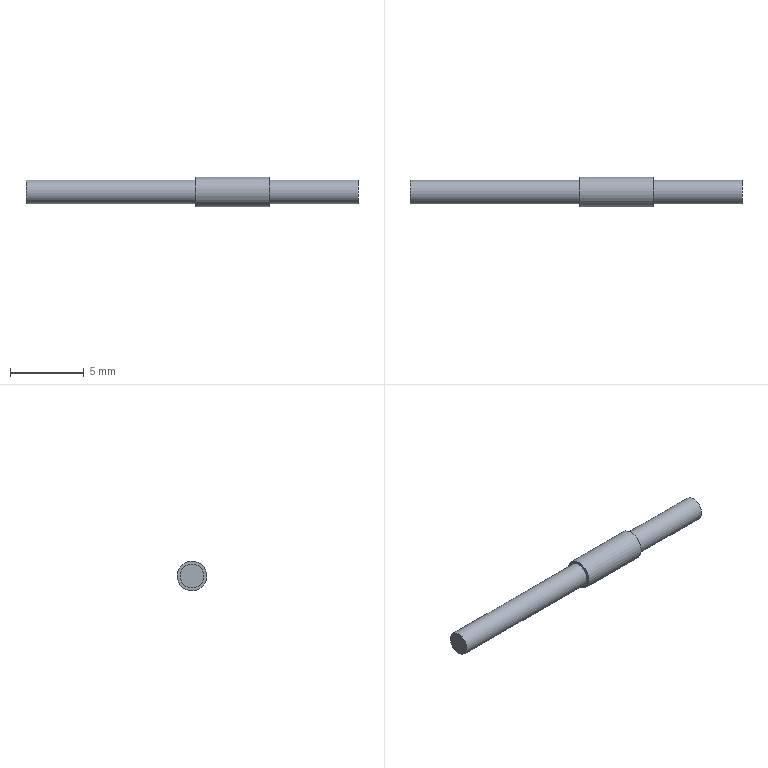Component | NX | BELT_SHAFT_2_2 | 1 solid | 7 faces | box 22.5 x 2 x 2 mm | volume 51 mm3 | plane 4 | cylinder 3 | commonest cylinder face diameters 1.6 x2 2 x1
STEP:
#1=CARTESIAN_POINT('',(0.,0.,0.));
#2=DIRECTION('',(0.,0.,1.));
#3=DIRECTION('',(1.,0.,0.));
#4=AXIS2_PLACEMENT_3D('',#1,#2,#3);
#5=CARTESIAN_POINT('',(-31.,-2.663,29.589));
#6=VERTEX_POINT('',#5);
#7=CARTESIAN_POINT('',(-31.,-3.575,30.));
#8=DIRECTION('',(1.,0.,0.));
#9=DIRECTION('',(0.,0.9116,-0.4111));
#10=AXIS2_PLACEMENT_3D('',#7,#8,#9);
#11=CIRCLE('',#10,1.);
#12=CARTESIAN_POINT('',(-36.,-3.575,30.));
#13=DIRECTION('',(1.,0.,0.));
#14=DIRECTION('',(0.,0.9116,-0.4111));
#15=AXIS2_PLACEMENT_3D('',#12,#13,#14);
#16=CYLINDRICAL_SURFACE('',#15,1.);
#17=CARTESIAN_POINT('',(0.,5.));
#18=DIRECTION('',(1.,0.));
#19=VECTOR('',#18,1.);
#20=LINE('',#17,#19);
#21=(GEOMETRIC_REPRESENTATION_CONTEXT(2)PARAMETRIC_REPRESENTATION_CONTEXT()REPRESENTATION_CONTEXT('',''));
#22=DEFINITIONAL_REPRESENTATION('',(#20),#21);
#23=PCURVE('',#16,#22);
#24=CARTESIAN_POINT('',(-31.,-3.986,29.088));
#25=DIRECTION('',(-1.,0.,0.));
#26=DIRECTION('',(0.,-0.9116,0.4111));
#27=AXIS2_PLACEMENT_3D('',#24,#25,#26);
#28=PLANE('',#27);
#29=CARTESIAN_POINT('',(-1.,1.));
#30=CARTESIAN_POINT('',(-1.,2.732));
#31=CARTESIAN_POINT('',(0.5,1.866));
#32=CARTESIAN_POINT('',(2.,1.));
#33=CARTESIAN_POINT('',(0.5,0.134));
#34=CARTESIAN_POINT('',(-1.,-0.7321));
#35=CARTESIAN_POINT('',(-1.,1.));
#36=(BOUNDED_CURVE()B_SPLINE_CURVE(2,(#29,#30,#31,#32,#33,#34,#35),.UNSPECIFIED.,.T.,.F.)B_SPLINE_CURVE_WITH_KNOTS((1,2,2,2,2,1),(-2.094,0.,2.094,4.189,6.283,8.378),.UNSPECIFIED.)CURVE()GEOMETRIC_REPRESENTATION_ITEM()RATIONAL_B_SPLINE_CURVE((1.,0.5,1.,0.5,1.,0.5,1.))REPRESENTATION_ITEM(''));
#37=(GEOMETRIC_REPRESENTATION_CONTEXT(2)PARAMETRIC_REPRESENTATION_CONTEXT()REPRESENTATION_CONTEXT('',''));
#38=DEFINITIONAL_REPRESENTATION('',(#36),#37);
#39=PCURVE('',#28,#38);
#40=SURFACE_CURVE('',#11,(#23,#39),.PCURVE_S1.);
#41=EDGE_CURVE('',#6,#6,#40,.T.);
#42=ORIENTED_EDGE('',*,*,#41,.F.);
#43=CARTESIAN_POINT('',(-36.,-2.663,29.589));
#44=VERTEX_POINT('',#43);
#45=CARTESIAN_POINT('',(-36.,-2.663,29.589));
#46=CARTESIAN_POINT('',(-31.,-2.663,29.589));
#47=B_SPLINE_CURVE_WITH_KNOTS('',1,(#45,#46),.UNSPECIFIED.,.F.,.F.,(2,2),(0.,5.),.PIECEWISE_BEZIER_KNOTS.);
#48=CARTESIAN_POINT('',(0.,0.));
#49=DIRECTION('',(0.,1.));
#50=VECTOR('',#49,1.);
#51=LINE('',#48,#50);
#52=(GEOMETRIC_REPRESENTATION_CONTEXT(2)PARAMETRIC_REPRESENTATION_CONTEXT()REPRESENTATION_CONTEXT('',''));
#53=DEFINITIONAL_REPRESENTATION('',(#51),#52);
#54=PCURVE('',#16,#53);
#55=CARTESIAN_POINT('',(6.283,0.));
#56=DIRECTION('',(0.,1.));
#57=VECTOR('',#56,1.);
#58=LINE('',#55,#57);
#59=(GEOMETRIC_REPRESENTATION_CONTEXT(2)PARAMETRIC_REPRESENTATION_CONTEXT()REPRESENTATION_CONTEXT('',''));
#60=DEFINITIONAL_REPRESENTATION('',(#58),#59);
#61=PCURVE('',#16,#60);
#62=SEAM_CURVE('',#47,(#54,#61),.PCURVE_S1.);
#63=EDGE_CURVE('',#44,#6,#62,.T.);
#64=ORIENTED_EDGE('',*,*,#63,.F.);
#65=CARTESIAN_POINT('',(-36.,-3.575,30.));
#66=DIRECTION('',(1.,0.,0.));
#67=DIRECTION('',(0.,0.9116,-0.4111));
#68=AXIS2_PLACEMENT_3D('',#65,#66,#67);
#69=CIRCLE('',#68,1.);
#70=CARTESIAN_POINT('',(0.,0.));
#71=DIRECTION('',(1.,0.));
#72=VECTOR('',#71,1.);
#73=LINE('',#70,#72);
#74=(GEOMETRIC_REPRESENTATION_CONTEXT(2)PARAMETRIC_REPRESENTATION_CONTEXT()REPRESENTATION_CONTEXT('',''));
#75=DEFINITIONAL_REPRESENTATION('',(#73),#74);
#76=PCURVE('',#16,#75);
#77=CARTESIAN_POINT('',(-36.,-3.904,29.271));
#78=DIRECTION('',(1.,0.,0.));
#79=DIRECTION('',(0.,0.9116,-0.4111));
#80=AXIS2_PLACEMENT_3D('',#77,#78,#79);
#81=PLANE('',#80);
#82=CARTESIAN_POINT('',(0.,0.8));
#83=DIRECTION('',(1.,0.));
#84=AXIS2_PLACEMENT_2D('',#82,#83);
#85=CIRCLE('',#84,1.);
#86=(GEOMETRIC_REPRESENTATION_CONTEXT(2)PARAMETRIC_REPRESENTATION_CONTEXT()REPRESENTATION_CONTEXT('',''));
#87=DEFINITIONAL_REPRESENTATION('',(#85),#86);
#88=PCURVE('',#81,#87);
#89=SURFACE_CURVE('',#69,(#76,#88),.PCURVE_S1.);
#90=EDGE_CURVE('',#44,#44,#89,.T.);
#91=ORIENTED_EDGE('',*,*,#90,.T.);
#92=ORIENTED_EDGE('',*,*,#63,.T.);
#93=EDGE_LOOP('',(#42,#64,#91,#92));
#94=FACE_BOUND('',#93,.T.);
#95=ADVANCED_FACE('',(#94),#16,.T.);
#96=CARTESIAN_POINT('',(-31.,-2.845,29.671));
#97=VERTEX_POINT('',#96);
#98=CARTESIAN_POINT('',(-31.,-3.575,30.));
#99=DIRECTION('',(1.,0.,0.));
#100=DIRECTION('',(0.,0.9116,-0.4111));
#101=AXIS2_PLACEMENT_3D('',#98,#99,#100);
#102=CIRCLE('',#101,0.8);
#103=CARTESIAN_POINT('',(-0.8,1.));
#104=CARTESIAN_POINT('',(-0.8,2.386));
#105=CARTESIAN_POINT('',(0.4,1.693));
#106=CARTESIAN_POINT('',(1.6,1.));
#107=CARTESIAN_POINT('',(0.4,0.3072));
#108=CARTESIAN_POINT('',(-0.8,-0.3856));
#109=CARTESIAN_POINT('',(-0.8,1.));
#110=(BOUNDED_CURVE()B_SPLINE_CURVE(2,(#103,#104,#105,#106,#107,#108,#109),.UNSPECIFIED.,.T.,.F.)B_SPLINE_CURVE_WITH_KNOTS((1,2,2,2,2,1),(-2.094,0.,2.094,4.189,6.283,8.378),.UNSPECIFIED.)CURVE()GEOMETRIC_REPRESENTATION_ITEM()RATIONAL_B_SPLINE_CURVE((1.,0.5,1.,0.5,1.,0.5,1.))REPRESENTATION_ITEM(''));
#111=(GEOMETRIC_REPRESENTATION_CONTEXT(2)PARAMETRIC_REPRESENTATION_CONTEXT()REPRESENTATION_CONTEXT('',''));
#112=DEFINITIONAL_REPRESENTATION('',(#110),#111);
#113=PCURVE('',#28,#112);
#114=CARTESIAN_POINT('',(-36.,-3.575,30.));
#115=DIRECTION('',(1.,0.,0.));
#116=DIRECTION('',(0.,0.9116,-0.4111));
#117=AXIS2_PLACEMENT_3D('',#114,#115,#116);
#118=CYLINDRICAL_SURFACE('',#117,0.8);
#119=CARTESIAN_POINT('',(0.,5.));
#120=DIRECTION('',(1.,0.));
#121=VECTOR('',#120,1.);
#122=LINE('',#119,#121);
#123=(GEOMETRIC_REPRESENTATION_CONTEXT(2)PARAMETRIC_REPRESENTATION_CONTEXT()REPRESENTATION_CONTEXT('',''));
#124=DEFINITIONAL_REPRESENTATION('',(#122),#123);
#125=PCURVE('',#118,#124);
#126=SURFACE_CURVE('',#102,(#113,#125),.PCURVE_S1.);
#127=EDGE_CURVE('',#97,#97,#126,.T.);
#128=ORIENTED_EDGE('',*,*,#127,.F.);
#129=EDGE_LOOP('',(#128));
#130=FACE_BOUND('',#129,.T.);
#131=ORIENTED_EDGE('',*,*,#41,.T.);
#132=EDGE_LOOP('',(#131));
#133=FACE_BOUND('',#132,.T.);
#134=ADVANCED_FACE('',(#130,#133),#28,.F.);
#135=CARTESIAN_POINT('',(-25.,-2.845,29.671));
#136=VERTEX_POINT('',#135);
#137=CARTESIAN_POINT('',(-25.,-3.575,30.));
#138=DIRECTION('',(1.,0.,0.));
#139=DIRECTION('',(0.,0.9116,-0.4111));
#140=AXIS2_PLACEMENT_3D('',#137,#138,#139);
#141=CIRCLE('',#140,0.8);
#142=CARTESIAN_POINT('',(0.,11.));
#143=DIRECTION('',(1.,0.));
#144=VECTOR('',#143,1.);
#145=LINE('',#142,#144);
#146=(GEOMETRIC_REPRESENTATION_CONTEXT(2)PARAMETRIC_REPRESENTATION_CONTEXT()REPRESENTATION_CONTEXT('',''));
#147=DEFINITIONAL_REPRESENTATION('',(#145),#146);
#148=PCURVE('',#118,#147);
#149=CARTESIAN_POINT('',(-25.,-3.904,29.271));
#150=DIRECTION('',(-1.,0.,0.));
#151=DIRECTION('',(0.,-0.9116,0.4111));
#152=AXIS2_PLACEMENT_3D('',#149,#150,#151);
#153=PLANE('',#152);
#154=CARTESIAN_POINT('',(-0.8,0.8));
#155=CARTESIAN_POINT('',(-0.8,2.186));
#156=CARTESIAN_POINT('',(0.4,1.493));
#157=CARTESIAN_POINT('',(1.6,0.8));
#158=CARTESIAN_POINT('',(0.4,0.1072));
#159=CARTESIAN_POINT('',(-0.8,-0.5856));
#160=CARTESIAN_POINT('',(-0.8,0.8));
#161=(BOUNDED_CURVE()B_SPLINE_CURVE(2,(#154,#155,#156,#157,#158,#159,#160),.UNSPECIFIED.,.T.,.F.)B_SPLINE_CURVE_WITH_KNOTS((1,2,2,2,2,1),(-2.094,0.,2.094,4.189,6.283,8.378),.UNSPECIFIED.)CURVE()GEOMETRIC_REPRESENTATION_ITEM()RATIONAL_B_SPLINE_CURVE((1.,0.5,1.,0.5,1.,0.5,1.))REPRESENTATION_ITEM(''));
#162=(GEOMETRIC_REPRESENTATION_CONTEXT(2)PARAMETRIC_REPRESENTATION_CONTEXT()REPRESENTATION_CONTEXT('',''));
#163=DEFINITIONAL_REPRESENTATION('',(#161),#162);
#164=PCURVE('',#153,#163);
#165=SURFACE_CURVE('',#141,(#148,#164),.PCURVE_S1.);
#166=EDGE_CURVE('',#136,#136,#165,.T.);
#167=ORIENTED_EDGE('',*,*,#166,.F.);
#168=CARTESIAN_POINT('',(-31.,-2.845,29.671));
#169=CARTESIAN_POINT('',(-25.,-2.845,29.671));
#170=B_SPLINE_CURVE_WITH_KNOTS('',1,(#168,#169),.UNSPECIFIED.,.F.,.F.,(2,2),(5.,11.),.PIECEWISE_BEZIER_KNOTS.);
#171=CARTESIAN_POINT('',(0.,0.));
#172=DIRECTION('',(0.,1.));
#173=VECTOR('',#172,1.);
#174=LINE('',#171,#173);
#175=(GEOMETRIC_REPRESENTATION_CONTEXT(2)PARAMETRIC_REPRESENTATION_CONTEXT()REPRESENTATION_CONTEXT('',''));
#176=DEFINITIONAL_REPRESENTATION('',(#174),#175);
#177=PCURVE('',#118,#176);
#178=CARTESIAN_POINT('',(6.283,0.));
#179=DIRECTION('',(0.,1.));
#180=VECTOR('',#179,1.);
#181=LINE('',#178,#180);
#182=(GEOMETRIC_REPRESENTATION_CONTEXT(2)PARAMETRIC_REPRESENTATION_CONTEXT()REPRESENTATION_CONTEXT('',''));
#183=DEFINITIONAL_REPRESENTATION('',(#181),#182);
#184=PCURVE('',#118,#183);
#185=SEAM_CURVE('',#170,(#177,#184),.PCURVE_S1.);
#186=EDGE_CURVE('',#97,#136,#185,.T.);
#187=ORIENTED_EDGE('',*,*,#186,.F.);
#188=ORIENTED_EDGE('',*,*,#127,.T.);
#189=ORIENTED_EDGE('',*,*,#186,.T.);
#190=EDGE_LOOP('',(#167,#187,#188,#189));
#191=FACE_BOUND('',#190,.T.);
#192=ADVANCED_FACE('',(#191),#118,.T.);
#193=ORIENTED_EDGE('',*,*,#166,.T.);
#194=EDGE_LOOP('',(#193));
#195=FACE_BOUND('',#194,.T.);
#196=ADVANCED_FACE('',(#195),#153,.F.);
#197=CARTESIAN_POINT('',(-47.5,-2.845,29.671));
#198=VERTEX_POINT('',#197);
#199=CARTESIAN_POINT('',(-47.5,-3.575,30.));
#200=DIRECTION('',(1.,0.,0.));
#201=DIRECTION('',(0.,0.9116,-0.4111));
#202=AXIS2_PLACEMENT_3D('',#199,#200,#201);
#203=CIRCLE('',#202,0.8);
#204=CARTESIAN_POINT('',(-47.5,-3.575,30.));
#205=DIRECTION('',(1.,0.,0.));
#206=DIRECTION('',(0.,0.9116,-0.4111));
#207=AXIS2_PLACEMENT_3D('',#204,#205,#206);
#208=PLANE('',#207);
#209=CARTESIAN_POINT('',(0.,0.));
#210=DIRECTION('',(1.,-0.));
#211=AXIS2_PLACEMENT_2D('',#209,#210);
#212=CIRCLE('',#211,0.8);
#213=(GEOMETRIC_REPRESENTATION_CONTEXT(2)PARAMETRIC_REPRESENTATION_CONTEXT()REPRESENTATION_CONTEXT('',''));
#214=DEFINITIONAL_REPRESENTATION('',(#212),#213);
#215=PCURVE('',#208,#214);
#216=CARTESIAN_POINT('',(-36.,-3.575,30.));
#217=DIRECTION('',(1.,0.,0.));
#218=DIRECTION('',(0.,0.9116,-0.4111));
#219=AXIS2_PLACEMENT_3D('',#216,#217,#218);
#220=CYLINDRICAL_SURFACE('',#219,0.8);
#221=CARTESIAN_POINT('',(0.,-11.5));
#222=DIRECTION('',(1.,0.));
#223=VECTOR('',#222,1.);
#224=LINE('',#221,#223);
#225=(GEOMETRIC_REPRESENTATION_CONTEXT(2)PARAMETRIC_REPRESENTATION_CONTEXT()REPRESENTATION_CONTEXT('',''));
#226=DEFINITIONAL_REPRESENTATION('',(#224),#225);
#227=PCURVE('',#220,#226);
#228=SURFACE_CURVE('',#203,(#215,#227),.PCURVE_S1.);
#229=EDGE_CURVE('',#198,#198,#228,.T.);
#230=ORIENTED_EDGE('',*,*,#229,.F.);
#231=EDGE_LOOP('',(#230));
#232=FACE_BOUND('',#231,.T.);
#233=ADVANCED_FACE('',(#232),#208,.F.);
#234=CARTESIAN_POINT('',(-36.,-2.845,29.671));
#235=VERTEX_POINT('',#234);
#236=CARTESIAN_POINT('',(-36.,-3.575,30.));
#237=DIRECTION('',(1.,0.,0.));
#238=DIRECTION('',(0.,0.9116,-0.4111));
#239=AXIS2_PLACEMENT_3D('',#236,#237,#238);
#240=CIRCLE('',#239,0.8);
#241=CARTESIAN_POINT('',(0.,0.));
#242=DIRECTION('',(1.,0.));
#243=VECTOR('',#242,1.);
#244=LINE('',#241,#243);
#245=(GEOMETRIC_REPRESENTATION_CONTEXT(2)PARAMETRIC_REPRESENTATION_CONTEXT()REPRESENTATION_CONTEXT('',''));
#246=DEFINITIONAL_REPRESENTATION('',(#244),#245);
#247=PCURVE('',#220,#246);
#248=CARTESIAN_POINT('',(0.,0.8));
#249=DIRECTION('',(1.,0.));
#250=AXIS2_PLACEMENT_2D('',#248,#249);
#251=CIRCLE('',#250,0.8);
#252=(GEOMETRIC_REPRESENTATION_CONTEXT(2)PARAMETRIC_REPRESENTATION_CONTEXT()REPRESENTATION_CONTEXT('',''));
#253=DEFINITIONAL_REPRESENTATION('',(#251),#252);
#254=PCURVE('',#81,#253);
#255=SURFACE_CURVE('',#240,(#247,#254),.PCURVE_S1.);
#256=EDGE_CURVE('',#235,#235,#255,.T.);
#257=ORIENTED_EDGE('',*,*,#256,.F.);
#258=CARTESIAN_POINT('',(-47.5,-2.845,29.671));
#259=CARTESIAN_POINT('',(-36.,-2.845,29.671));
#260=B_SPLINE_CURVE_WITH_KNOTS('',1,(#258,#259),.UNSPECIFIED.,.F.,.F.,(2,2),(-11.5,0.),.PIECEWISE_BEZIER_KNOTS.);
#261=CARTESIAN_POINT('',(0.,0.));
#262=DIRECTION('',(0.,1.));
#263=VECTOR('',#262,1.);
#264=LINE('',#261,#263);
#265=(GEOMETRIC_REPRESENTATION_CONTEXT(2)PARAMETRIC_REPRESENTATION_CONTEXT()REPRESENTATION_CONTEXT('',''));
#266=DEFINITIONAL_REPRESENTATION('',(#264),#265);
#267=PCURVE('',#220,#266);
#268=CARTESIAN_POINT('',(6.283,0.));
#269=DIRECTION('',(0.,1.));
#270=VECTOR('',#269,1.);
#271=LINE('',#268,#270);
#272=(GEOMETRIC_REPRESENTATION_CONTEXT(2)PARAMETRIC_REPRESENTATION_CONTEXT()REPRESENTATION_CONTEXT('',''));
#273=DEFINITIONAL_REPRESENTATION('',(#271),#272);
#274=PCURVE('',#220,#273);
#275=SEAM_CURVE('',#260,(#267,#274),.PCURVE_S1.);
#276=EDGE_CURVE('',#198,#235,#275,.T.);
#277=ORIENTED_EDGE('',*,*,#276,.F.);
#278=ORIENTED_EDGE('',*,*,#229,.T.);
#279=ORIENTED_EDGE('',*,*,#276,.T.);
#280=EDGE_LOOP('',(#257,#277,#278,#279));
#281=FACE_BOUND('',#280,.T.);
#282=ADVANCED_FACE('',(#281),#220,.T.);
#283=ORIENTED_EDGE('',*,*,#90,.F.);
#284=EDGE_LOOP('',(#283));
#285=FACE_BOUND('',#284,.T.);
#286=ORIENTED_EDGE('',*,*,#256,.T.);
#287=EDGE_LOOP('',(#286));
#288=FACE_BOUND('',#287,.T.);
#289=ADVANCED_FACE('',(#285,#288),#81,.F.);
#290=CLOSED_SHELL('',(#95,#134,#192,#196,#233,#282,#289));
#291=MANIFOLD_SOLID_BREP('',#290);
#292=(LENGTH_UNIT()NAMED_UNIT(*)SI_UNIT(.MILLI.,.METRE.));
#293=UNCERTAINTY_MEASURE_WITH_UNIT(LENGTH_MEASURE(0.00001),#292,'','');
#294=(NAMED_UNIT(*)PLANE_ANGLE_UNIT()SI_UNIT($,.RADIAN.));
#295=(NAMED_UNIT(*)SI_UNIT($,.STERADIAN.)SOLID_ANGLE_UNIT());
#296=(GEOMETRIC_REPRESENTATION_CONTEXT(3)GLOBAL_UNCERTAINTY_ASSIGNED_CONTEXT((#293))GLOBAL_UNIT_ASSIGNED_CONTEXT((#292,#294,#295))REPRESENTATION_CONTEXT('',''));
#297=ADVANCED_BREP_SHAPE_REPRESENTATION('',(#4,#291),#296);